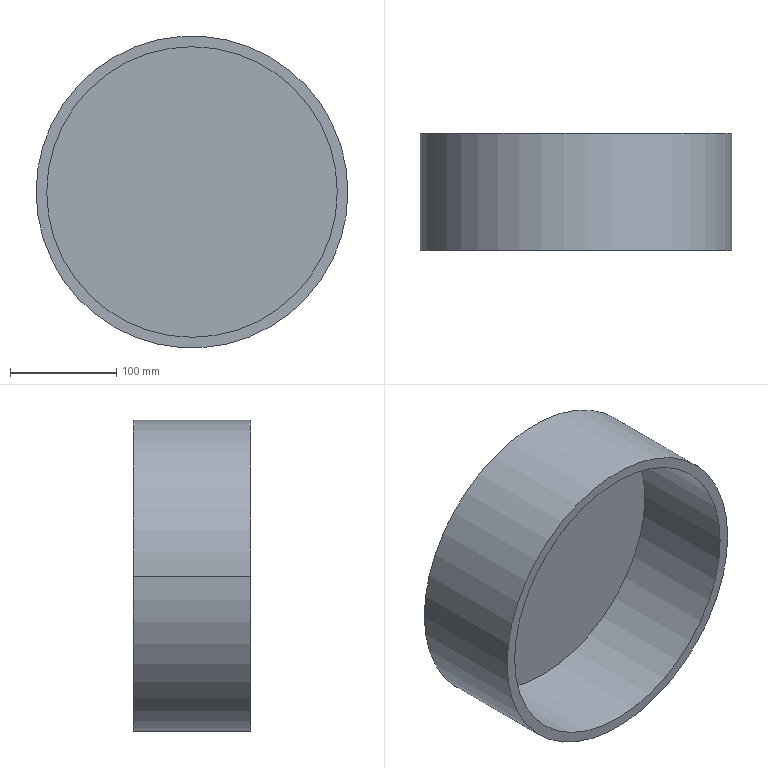Component | SolidWorks | Cap-1 | 1 solid | 7 faces | box 293 x 110 x 293 mm | volume 1563327 mm3 | cylinder 4 | plane 3 | commonest cylinder face diameters 273 x2 293 x2
build123d program:
from build123d import *

# Parameters (mm, degrees)
SKETCH1_R           = 146.5
SKETCH1_R_2         = 136.5
BOSS_EXTRUDE1_DEPTH = 100
BOSS_EXTRUDE2_START = 10
SKETCH2_R           = 146.5
BOSS_EXTRUDE2_DEPTH = 10


with BuildPart() as part:
    # Sketch1 → Boss-Extrude1 (new body)
    with BuildSketch(Plane.XY):
        Circle(SKETCH1_R)
        Circle(SKETCH1_R_2, mode=Mode.SUBTRACT)
    extrude(amount=-BOSS_EXTRUDE1_DEPTH)

    # Sketch2 → Boss-Extrude2 (add)
    with BuildSketch(Plane.XY.offset(BOSS_EXTRUDE2_START)):
        Circle(SKETCH2_R)
    extrude(amount=-BOSS_EXTRUDE2_DEPTH)


solid = part.part

# Placed as in the assembly
solid = solid.moved(Location((0, 8020, 0), (-90, 0, 0)))
STEP:
#1=COLOUR_RGB('',0.7922,0.8196,0.9333);
#2=FILL_AREA_STYLE_COLOUR('',#1);
#3=FILL_AREA_STYLE('',(#2));
#4=SURFACE_STYLE_FILL_AREA(#3);
#5=SURFACE_SIDE_STYLE('',(#4));
#6=SURFACE_STYLE_USAGE(.BOTH.,#5);
#7=PRESENTATION_STYLE_ASSIGNMENT((#6));
#8=CARTESIAN_POINT('',(-5.374,311.811,-0.01261));
#9=VERTEX_POINT('',#8);
#10=CARTESIAN_POINT('',(5.374,311.811,0.01261));
#11=VERTEX_POINT('',#10);
#12=CARTESIAN_POINT('',(0.,311.811,0.));
#13=DIRECTION('',(0.,1.,0.));
#14=DIRECTION('',(1.,0.,0.002347));
#15=AXIS2_PLACEMENT_3D('',#12,#13,#14);
#16=CIRCLE('',#15,5.374);
#17=EDGE_CURVE('',#9,#11,#16,.T.);
#18=ORIENTED_EDGE('',*,*,#17,.F.);
#19=CARTESIAN_POINT('',(-5.374,315.748,-0.01261));
#20=VERTEX_POINT('',#19);
#21=CARTESIAN_POINT('',(-5.374,311.811,-0.01261));
#22=DIRECTION('',(0.,1.,0.));
#23=VECTOR('',#22,39.37);
#24=LINE('',#21,#23);
#25=EDGE_CURVE('',#9,#20,#24,.T.);
#26=ORIENTED_EDGE('',*,*,#25,.T.);
#27=CARTESIAN_POINT('',(5.374,315.748,0.01261));
#28=VERTEX_POINT('',#27);
#29=CARTESIAN_POINT('',(0.,315.748,0.));
#30=DIRECTION('',(0.,1.,0.));
#31=DIRECTION('',(1.,0.,0.002347));
#32=AXIS2_PLACEMENT_3D('',#29,#30,#31);
#33=CIRCLE('',#32,5.374);
#34=EDGE_CURVE('',#20,#28,#33,.T.);
#35=ORIENTED_EDGE('',*,*,#34,.T.);
#36=CARTESIAN_POINT('',(5.374,311.811,0.01261));
#37=DIRECTION('',(0.,1.,0.));
#38=VECTOR('',#37,39.37);
#39=LINE('',#36,#38);
#40=EDGE_CURVE('',#11,#28,#39,.T.);
#41=ORIENTED_EDGE('',*,*,#40,.F.);
#42=EDGE_LOOP('',(#18,#26,#35,#41));
#43=FACE_OUTER_BOUND('',#42,.T.);
#44=CARTESIAN_POINT('',(0.,311.811,0.));
#45=DIRECTION('',(0.,1.,0.));
#46=DIRECTION('',(1.,0.,0.002347));
#47=AXIS2_PLACEMENT_3D('',#44,#45,#46);
#48=CYLINDRICAL_SURFACE('',#47,5.374);
#49=ADVANCED_FACE('',(#43),#48,.F.);
#50=CARTESIAN_POINT('',(5.768,311.811,0.01354));
#51=VERTEX_POINT('',#50);
#52=CARTESIAN_POINT('',(-5.768,311.811,-0.01354));
#53=VERTEX_POINT('',#52);
#54=CARTESIAN_POINT('',(0.,311.811,0.));
#55=DIRECTION('',(0.,1.,0.));
#56=DIRECTION('',(1.,0.,0.002347));
#57=AXIS2_PLACEMENT_3D('',#54,#55,#56);
#58=CIRCLE('',#57,5.768);
#59=EDGE_CURVE('',#51,#53,#58,.T.);
#60=ORIENTED_EDGE('',*,*,#59,.T.);
#61=CARTESIAN_POINT('',(-5.768,316.142,-0.01354));
#62=VERTEX_POINT('',#61);
#63=CARTESIAN_POINT('',(-5.768,311.811,-0.01354));
#64=DIRECTION('',(0.,1.,0.));
#65=VECTOR('',#64,39.37);
#66=LINE('',#63,#65);
#67=EDGE_CURVE('',#53,#62,#66,.T.);
#68=ORIENTED_EDGE('',*,*,#67,.T.);
#69=CARTESIAN_POINT('',(5.768,316.142,0.01354));
#70=VERTEX_POINT('',#69);
#71=CARTESIAN_POINT('',(0.,316.142,0.));
#72=DIRECTION('',(0.,1.,0.));
#73=DIRECTION('',(1.,0.,0.002347));
#74=AXIS2_PLACEMENT_3D('',#71,#72,#73);
#75=CIRCLE('',#74,5.768);
#76=EDGE_CURVE('',#70,#62,#75,.T.);
#77=ORIENTED_EDGE('',*,*,#76,.F.);
#78=CARTESIAN_POINT('',(5.768,311.811,0.01354));
#79=DIRECTION('',(0.,1.,0.));
#80=VECTOR('',#79,39.37);
#81=LINE('',#78,#80);
#82=EDGE_CURVE('',#51,#70,#81,.T.);
#83=ORIENTED_EDGE('',*,*,#82,.F.);
#84=EDGE_LOOP('',(#60,#68,#77,#83));
#85=FACE_OUTER_BOUND('',#84,.T.);
#86=CARTESIAN_POINT('',(0.,311.811,0.));
#87=DIRECTION('',(0.,1.,0.));
#88=DIRECTION('',(1.,0.,0.002347));
#89=AXIS2_PLACEMENT_3D('',#86,#87,#88);
#90=CYLINDRICAL_SURFACE('',#89,5.768);
#91=ADVANCED_FACE('',(#85),#90,.T.);
#92=ORIENTED_EDGE('',*,*,#67,.F.);
#93=CARTESIAN_POINT('',(0.,311.811,0.));
#94=DIRECTION('',(0.,1.,0.));
#95=DIRECTION('',(1.,0.,0.002347));
#96=AXIS2_PLACEMENT_3D('',#93,#94,#95);
#97=CIRCLE('',#96,5.768);
#98=EDGE_CURVE('',#53,#51,#97,.T.);
#99=ORIENTED_EDGE('',*,*,#98,.T.);
#100=ORIENTED_EDGE('',*,*,#82,.T.);
#101=CARTESIAN_POINT('',(0.,316.142,0.));
#102=DIRECTION('',(0.,1.,0.));
#103=DIRECTION('',(1.,0.,0.002347));
#104=AXIS2_PLACEMENT_3D('',#101,#102,#103);
#105=CIRCLE('',#104,5.768);
#106=EDGE_CURVE('',#62,#70,#105,.T.);
#107=ORIENTED_EDGE('',*,*,#106,.F.);
#108=EDGE_LOOP('',(#92,#99,#100,#107));
#109=FACE_OUTER_BOUND('',#108,.T.);
#110=CARTESIAN_POINT('',(0.,311.811,0.));
#111=DIRECTION('',(0.,1.,0.));
#112=DIRECTION('',(1.,0.,0.002347));
#113=AXIS2_PLACEMENT_3D('',#110,#111,#112);
#114=CYLINDRICAL_SURFACE('',#113,5.768);
#115=ADVANCED_FACE('',(#109),#114,.T.);
#116=CARTESIAN_POINT('',(0.,311.811,0.));
#117=DIRECTION('',(0.,1.,0.));
#118=DIRECTION('',(1.,0.,0.002347));
#119=AXIS2_PLACEMENT_3D('',#116,#117,#118);
#120=CIRCLE('',#119,5.374);
#121=EDGE_CURVE('',#11,#9,#120,.T.);
#122=ORIENTED_EDGE('',*,*,#121,.T.);
#123=ORIENTED_EDGE('',*,*,#17,.T.);
#124=EDGE_LOOP('',(#122,#123));
#125=FACE_BOUND('',#124,.T.);
#126=ORIENTED_EDGE('',*,*,#59,.F.);
#127=ORIENTED_EDGE('',*,*,#98,.F.);
#128=EDGE_LOOP('',(#126,#127));
#129=FACE_OUTER_BOUND('',#128,.T.);
#130=CARTESIAN_POINT('',(0.,311.811,0.));
#131=DIRECTION('',(0.,1.,0.));
#132=DIRECTION('',(1.,0.,0.002347));
#133=AXIS2_PLACEMENT_3D('',#130,#131,#132);
#134=PLANE('',#133);
#135=ADVANCED_FACE('',(#125,#129),#134,.F.);
#136=ORIENTED_EDGE('',*,*,#25,.F.);
#137=ORIENTED_EDGE('',*,*,#121,.F.);
#138=ORIENTED_EDGE('',*,*,#40,.T.);
#139=CARTESIAN_POINT('',(0.,315.748,0.));
#140=DIRECTION('',(0.,1.,0.));
#141=DIRECTION('',(1.,0.,0.002347));
#142=AXIS2_PLACEMENT_3D('',#139,#140,#141);
#143=CIRCLE('',#142,5.374);
#144=EDGE_CURVE('',#28,#20,#143,.T.);
#145=ORIENTED_EDGE('',*,*,#144,.T.);
#146=EDGE_LOOP('',(#136,#137,#138,#145));
#147=FACE_OUTER_BOUND('',#146,.T.);
#148=CARTESIAN_POINT('',(0.,311.811,0.));
#149=DIRECTION('',(0.,1.,0.));
#150=DIRECTION('',(1.,0.,0.002347));
#151=AXIS2_PLACEMENT_3D('',#148,#149,#150);
#152=CYLINDRICAL_SURFACE('',#151,5.374);
#153=ADVANCED_FACE('',(#147),#152,.F.);
#154=ORIENTED_EDGE('',*,*,#144,.F.);
#155=ORIENTED_EDGE('',*,*,#34,.F.);
#156=EDGE_LOOP('',(#154,#155));
#157=FACE_OUTER_BOUND('',#156,.T.);
#158=CARTESIAN_POINT('',(0.,315.748,0.));
#159=DIRECTION('',(0.,1.,0.));
#160=DIRECTION('',(1.,0.,0.002347));
#161=AXIS2_PLACEMENT_3D('',#158,#159,#160);
#162=PLANE('',#161);
#163=ADVANCED_FACE('',(#157),#162,.F.);
#164=ORIENTED_EDGE('',*,*,#76,.T.);
#165=ORIENTED_EDGE('',*,*,#106,.T.);
#166=EDGE_LOOP('',(#164,#165));
#167=FACE_OUTER_BOUND('',#166,.T.);
#168=CARTESIAN_POINT('',(0.,316.142,0.));
#169=DIRECTION('',(0.,1.,0.));
#170=DIRECTION('',(1.,0.,0.002347));
#171=AXIS2_PLACEMENT_3D('',#168,#169,#170);
#172=PLANE('',#171);
#173=ADVANCED_FACE('',(#167),#172,.T.);
#174=CLOSED_SHELL('',(#49,#91,#115,#135,#153,#163,#173));
#175=MANIFOLD_SOLID_BREP('',#174);
#176=STYLED_ITEM('',(#7),#175);
#177=PRESENTATION_LAYER_ASSIGNMENT('','',(#176));
#178=CARTESIAN_POINT('',(0.,0.,0.));
#179=DIRECTION('',(0.,0.,1.));
#180=DIRECTION('',(1.,0.,0.));
#181=AXIS2_PLACEMENT_3D('',#178,#179,#180);
#182=(LENGTH_UNIT()NAMED_UNIT(*)SI_UNIT($,.METRE.));
#183=LENGTH_MEASURE_WITH_UNIT(LENGTH_MEASURE(0.0254),#182);
#184=DIMENSIONAL_EXPONENTS(1.,0.,0.,0.,0.,0.,0.);
#185=(CONVERSION_BASED_UNIT('',#183)LENGTH_UNIT()NAMED_UNIT(#184));
#186=UNCERTAINTY_MEASURE_WITH_UNIT(LENGTH_MEASURE(0.00001),#185,'','');
#187=(NAMED_UNIT(*)PLANE_ANGLE_UNIT()SI_UNIT($,.RADIAN.));
#188=(NAMED_UNIT(*)SI_UNIT($,.STERADIAN.)SOLID_ANGLE_UNIT());
#189=(GEOMETRIC_REPRESENTATION_CONTEXT(3)GLOBAL_UNCERTAINTY_ASSIGNED_CONTEXT((#186))GLOBAL_UNIT_ASSIGNED_CONTEXT((#185,#187,#188))REPRESENTATION_CONTEXT('',''));
#190=ADVANCED_BREP_SHAPE_REPRESENTATION('',(#175,#181),#189);
#191=(LENGTH_UNIT()NAMED_UNIT(*)SI_UNIT($,.METRE.));
#192=LENGTH_MEASURE_WITH_UNIT(LENGTH_MEASURE(0.0254),#191);
#193=DIMENSIONAL_EXPONENTS(1.,0.,0.,0.,0.,0.,0.);
#194=(CONVERSION_BASED_UNIT('',#192)LENGTH_UNIT()NAMED_UNIT(#193));
#195=UNCERTAINTY_MEASURE_WITH_UNIT(LENGTH_MEASURE(0.00001),#194,'','');
#196=(NAMED_UNIT(*)PLANE_ANGLE_UNIT()SI_UNIT($,.RADIAN.));
#197=(NAMED_UNIT(*)SI_UNIT($,.STERADIAN.)SOLID_ANGLE_UNIT());
#198=(GEOMETRIC_REPRESENTATION_CONTEXT(3)GLOBAL_UNCERTAINTY_ASSIGNED_CONTEXT((#195))GLOBAL_UNIT_ASSIGNED_CONTEXT((#194,#196,#197))REPRESENTATION_CONTEXT('',''));
#199=MECHANICAL_DESIGN_GEOMETRIC_PRESENTATION_REPRESENTATION('',(#176),#198);